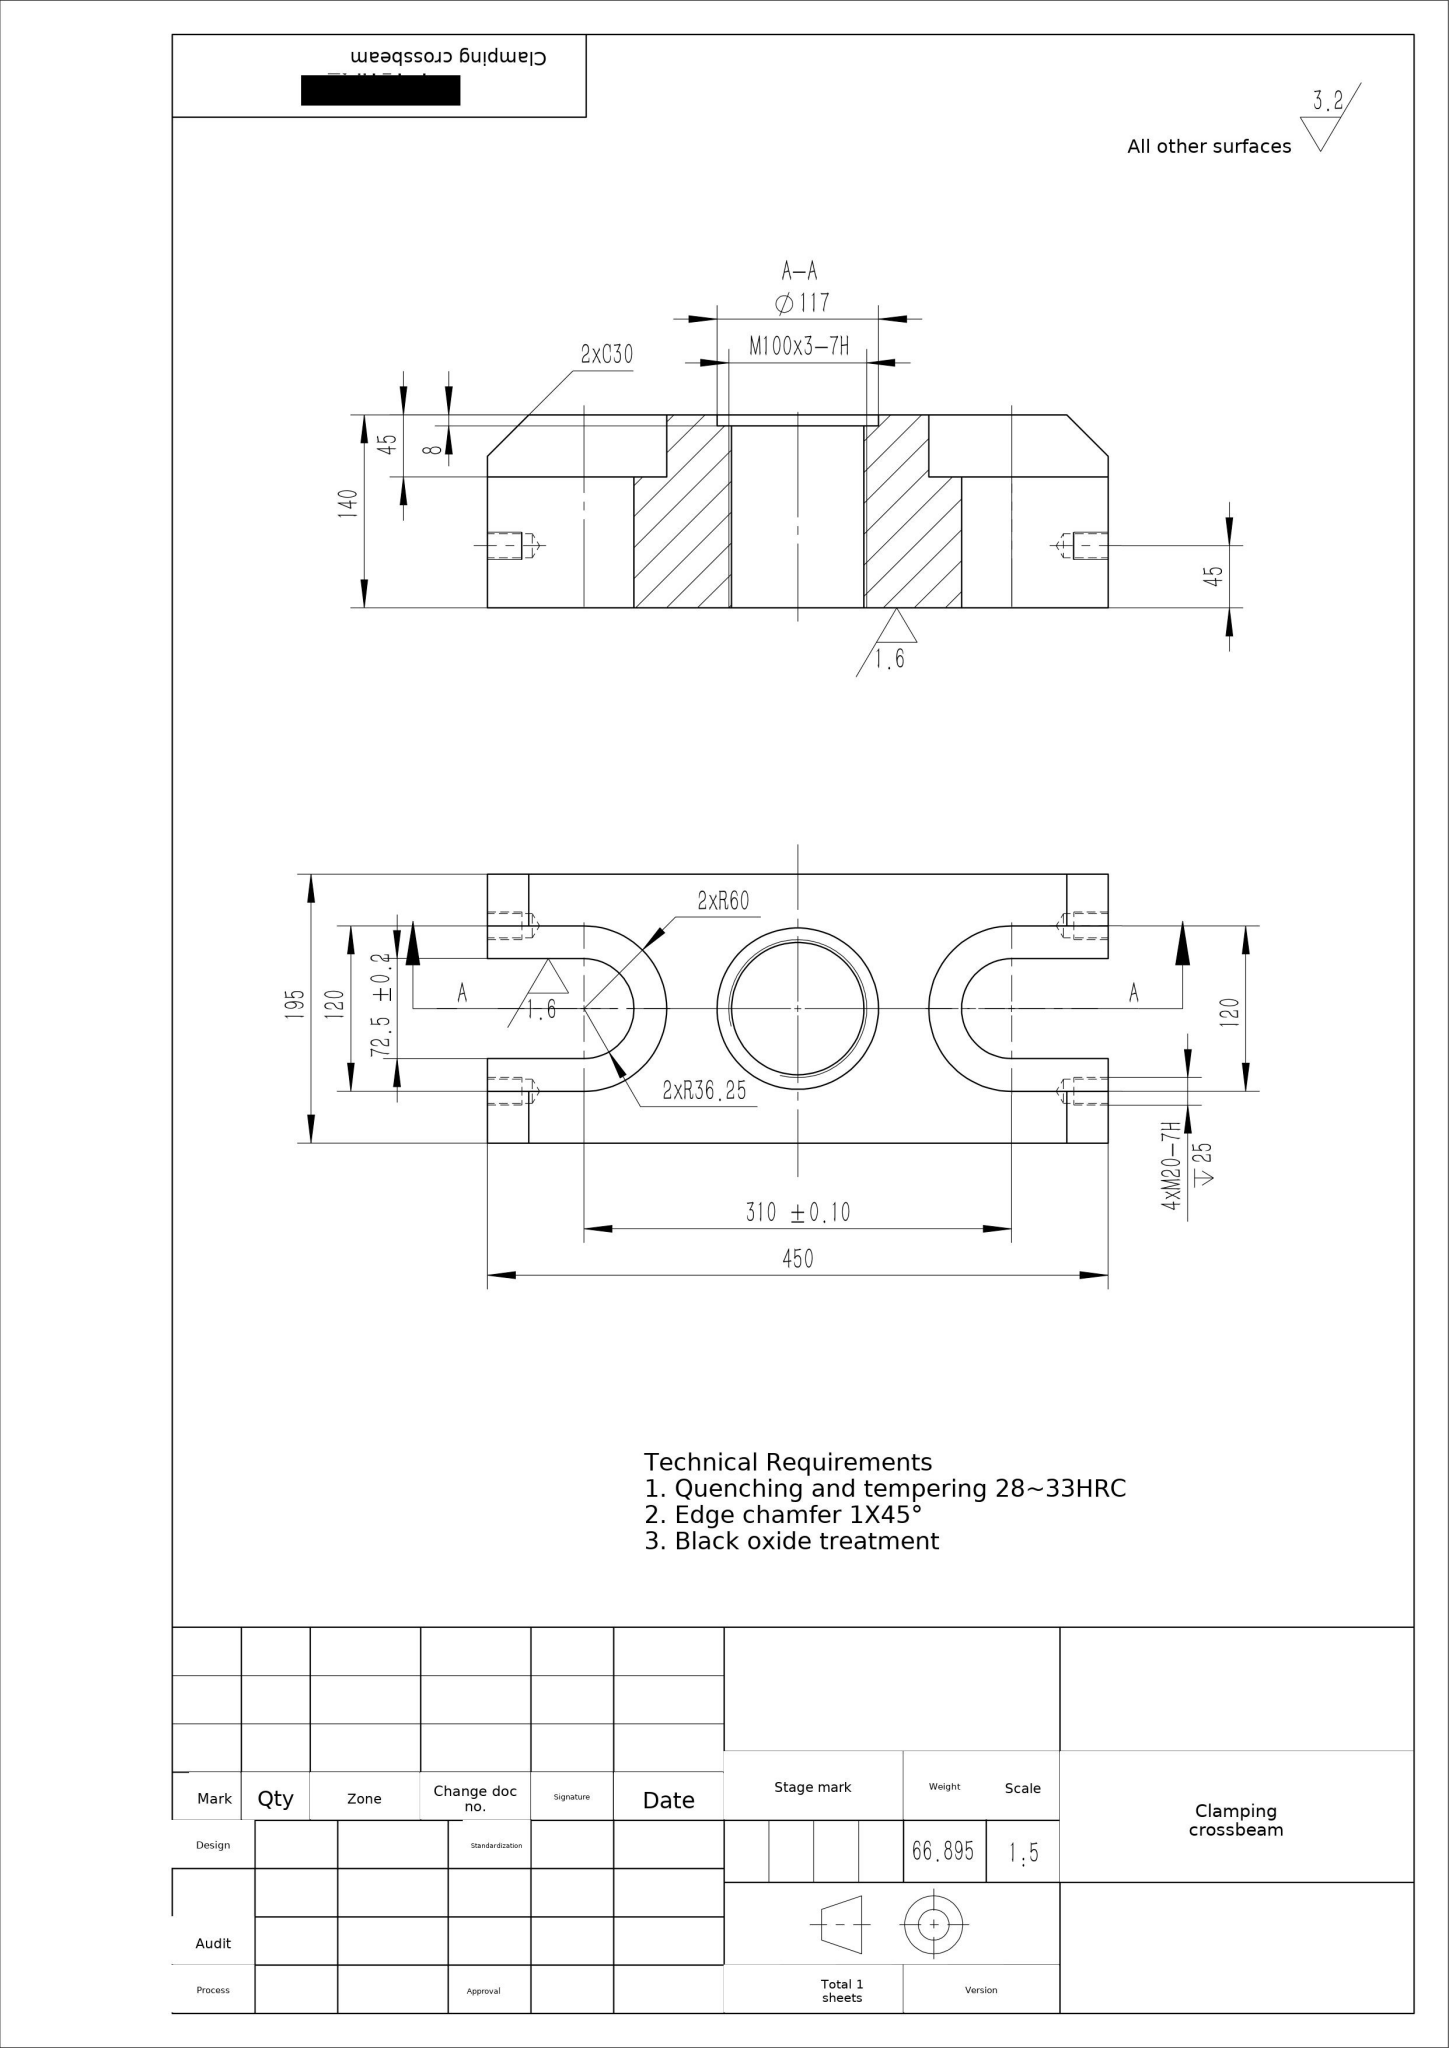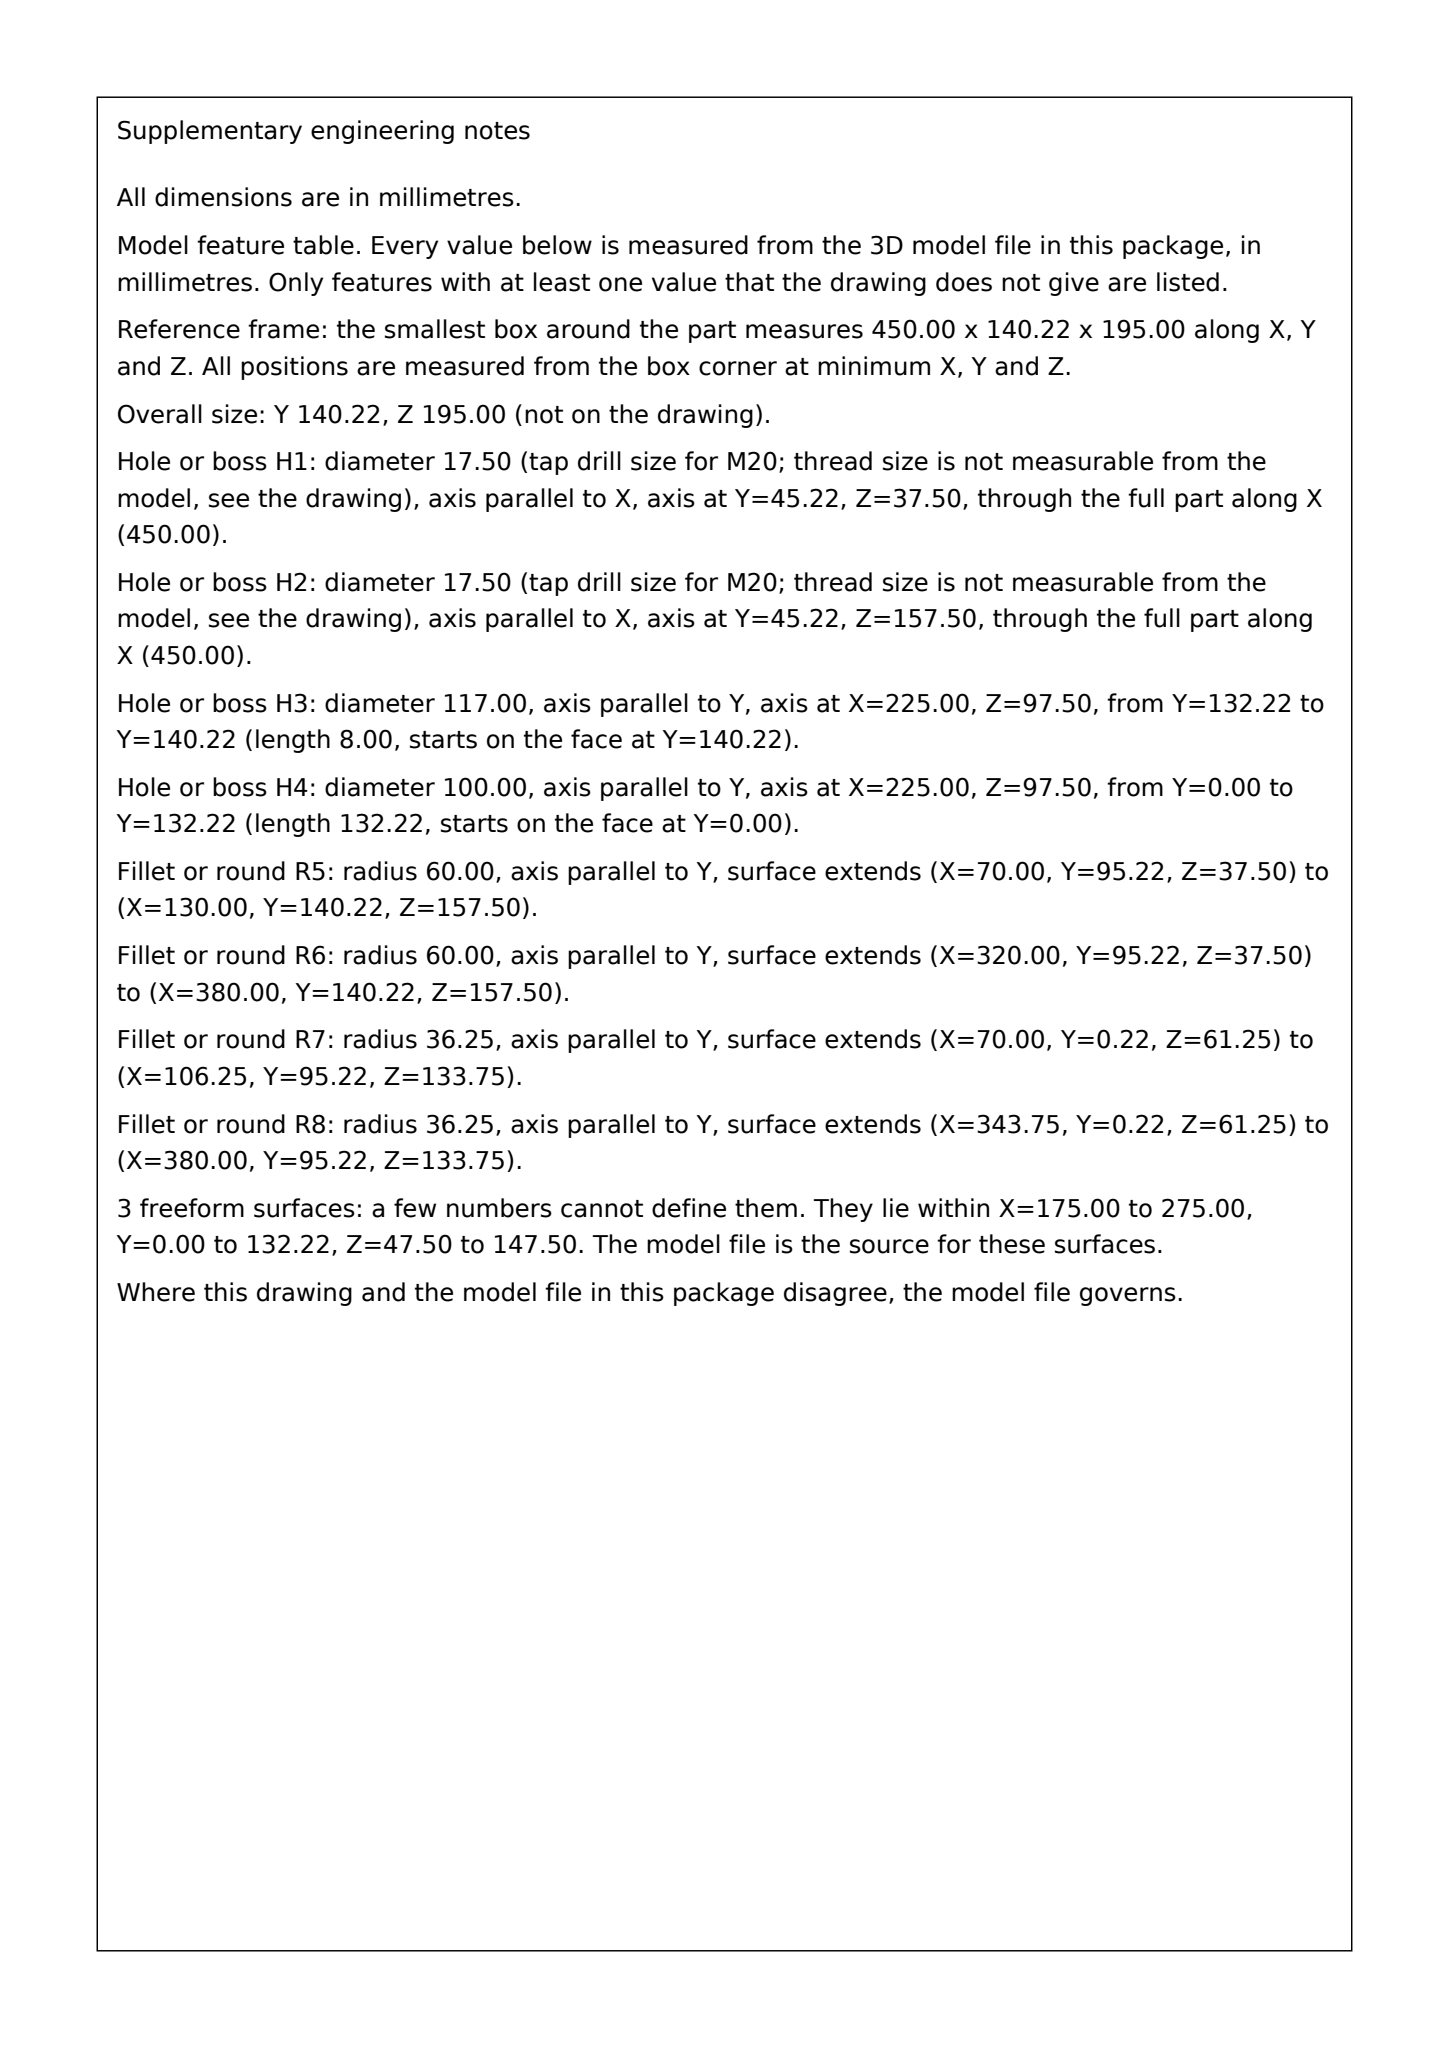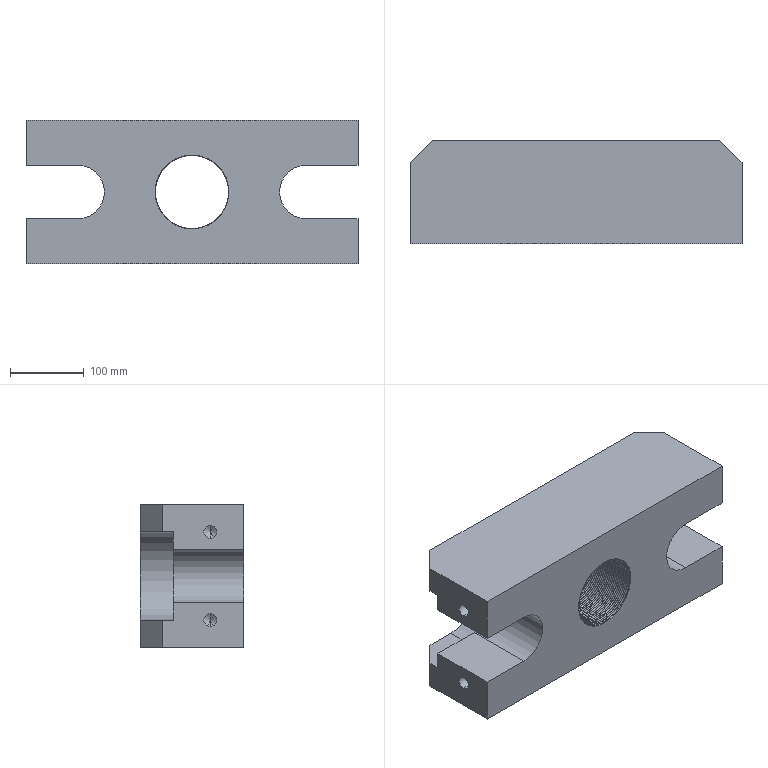Part | SolidWorks | mm | 1 solid | 142 faces | box 450 x 140.22 x 195 mm | volume 8440389 mm3 | cylinder 106 | plane 25 | cone 8 | spline 3 | commonest cylinder face diameters 100 x92 17.5 x8 117 x2 72.5 x2 120 x2